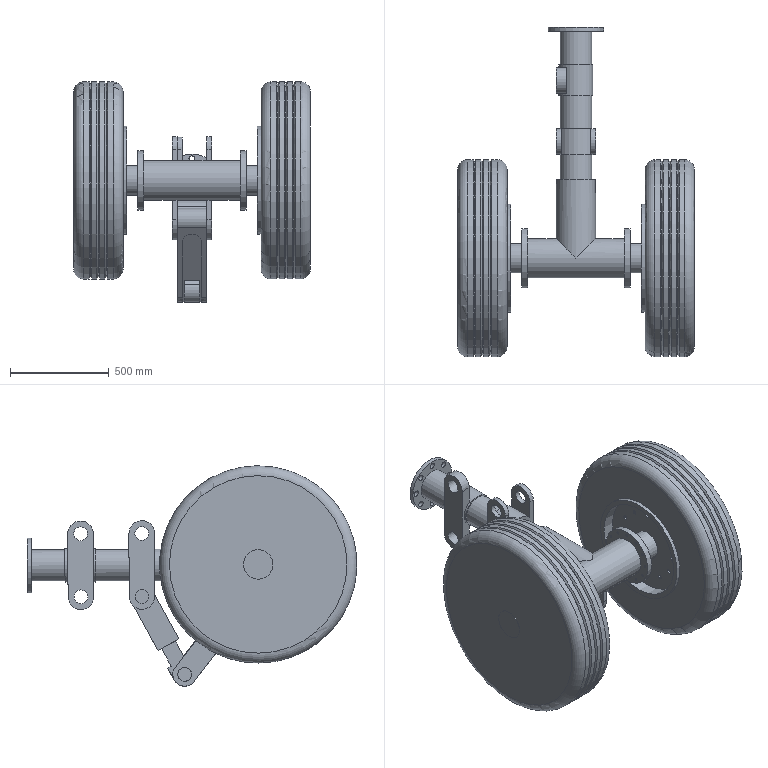Assembly | NX | mm | 12 component files | 12 solids | 228 faces | box 1200.7 x 1670.67 x 1117.5 mm | volume 437227469 mm3 | cylinder 123 | plane 88 | cone 12 | torus 4 | spline 1 | commonest cylinder face diameters 12 x24 20 x24 70 x16 1000 x8 30 x8 200 x6 150 x6 95 x6
Bill of materials:
unnamed part 1 | 1 |  | Plain solid cylinder with flat ends; length roughly twice the diameter.
unnamed part 2 | 1 |  | Helical coil of round-section wire, about 10 turns at constant coil diameter and roughly even pitch, with plain cut ends.
unnamed part 3 | 2 |  | Thick circular disc or wheel with a small central through-hole, rounded outer edges, and three shallow circumferential grooves around the rim; a thin, smaller-diameter raised step appears on one face.
unnamed part 4 | 1 |  | Elongated flat link with rounded ends and a through-hole at each end. The width is stepped: a wider section and a narrower section, with small rectangular notches/shoulders at the transition. There is a curved arc-shaped recess or slot near the wider end.
unnamed part 5 | 2 |  | Plain solid cylinder with flat ends; length roughly three times the diameter.
unnamed part 6 | 1 |  | Tee-shaped tubular body: a straight main cylindrical run with two large circular flanges, each carrying a ring of small holes on a bolt circle, and a perpendicular cylindrical branch joined midway. A flat plate tab with a rounded end and a single round hole projects below the run.
unnamed part 7 | 1 |  | Straight bar with fully rounded ends and a through-hole at each end. A rectangular open slot at one end splits it into two tines, forming a fork/clevis-like end.
unnamed part 8 | 1 |  | Cylindrical shaft or tube body with a circular flange at one end carrying a ring of holes, a plain flat opposite end, and a slightly larger collar band. Two flat lug plates with rounded ends and two holes each pass crosswise through the body at two axial positions.
unnamed part 9 | 2 |  | Thin flat annular disc with a large central hole and 12 small holes evenly spaced on a bolt circle.
Mates:
1. touch align | wheel 1 face | wheel 2 face
2. touch align | brake_pad 2 face | wheel 1 face
3. touch align | brake_pad 2 face | wheel 1 face
4. touch align | brake_pad 1 face | wheel 2 face
5. touch align | axle 1 face | wheel 2 face
6. touch align | column 1 face | axle 1 face
7. touch align | column 1 face | axle 1 face
8. touch align | upper_hyd_rod 1 face | column 1 face
9. touch align | upper_hyd_rod 1 face | column 1 face
10. touch align | lower_hyd_rod 1 face | axle 1 face
11. touch align | lower_hyd_rod 1 face | axle 1 face
12. touch align | upper_hyd_rod 1 face | lower_hyd_rod 1 face
13. touch align | upper_hyd_rod 1 face | column 1 face
14. concentric | shaft_pin_70_150 1 edge | lower_hyd_rod 1 edge
15. concentric | shaft_pin_70_200 1 edge | column 1 edge
16. concentric | shaft_pin_70_200 2 edge | axle 1 edge